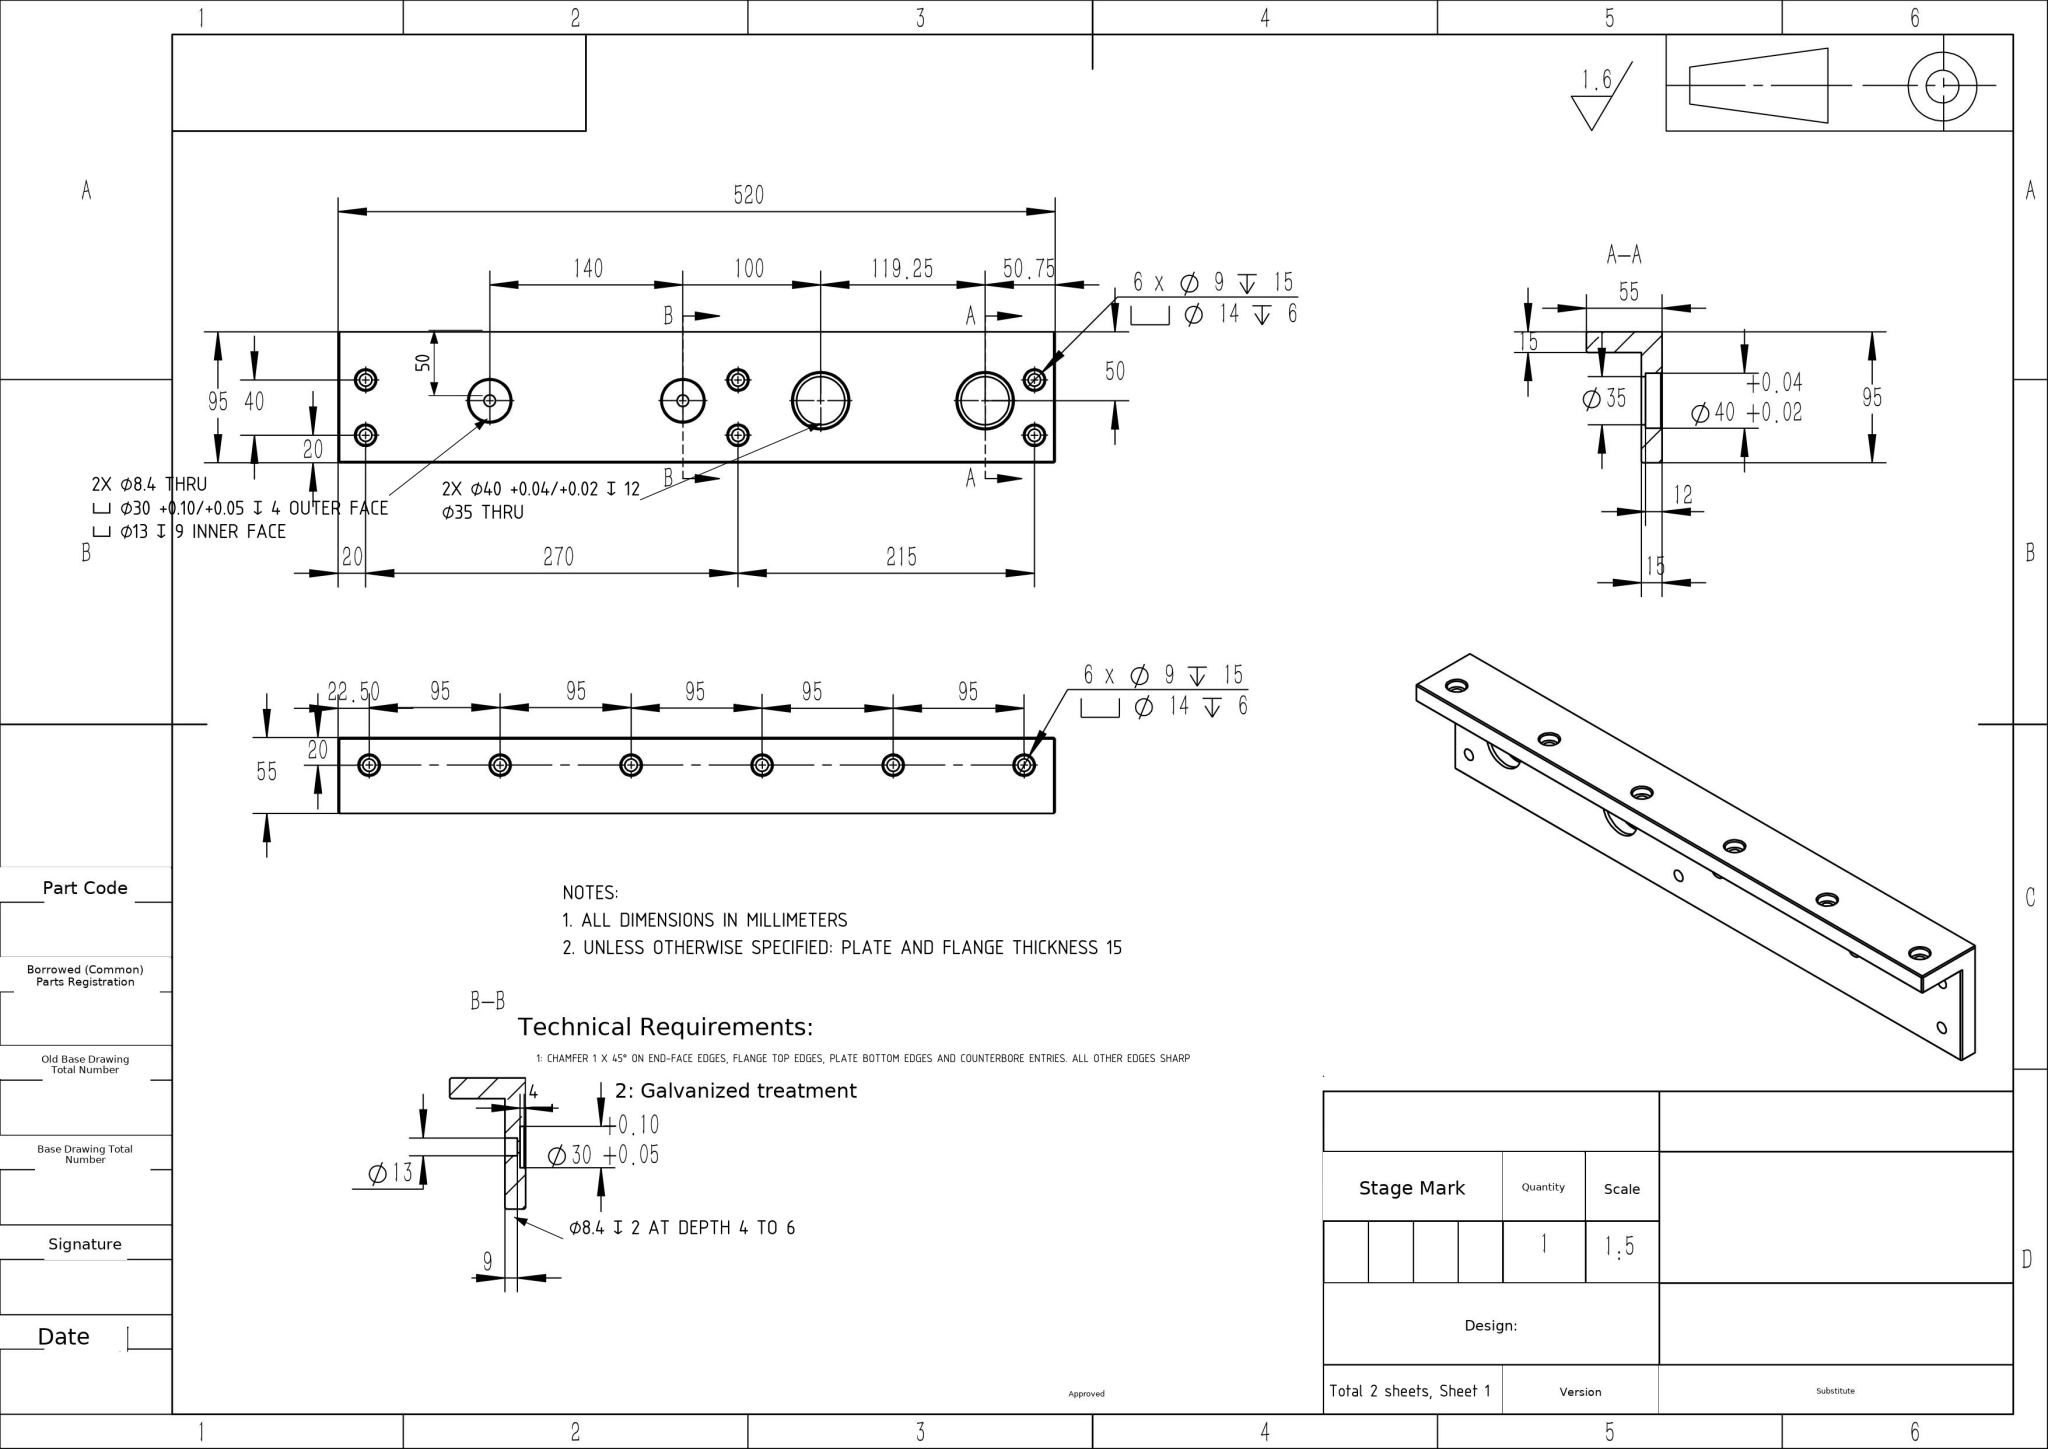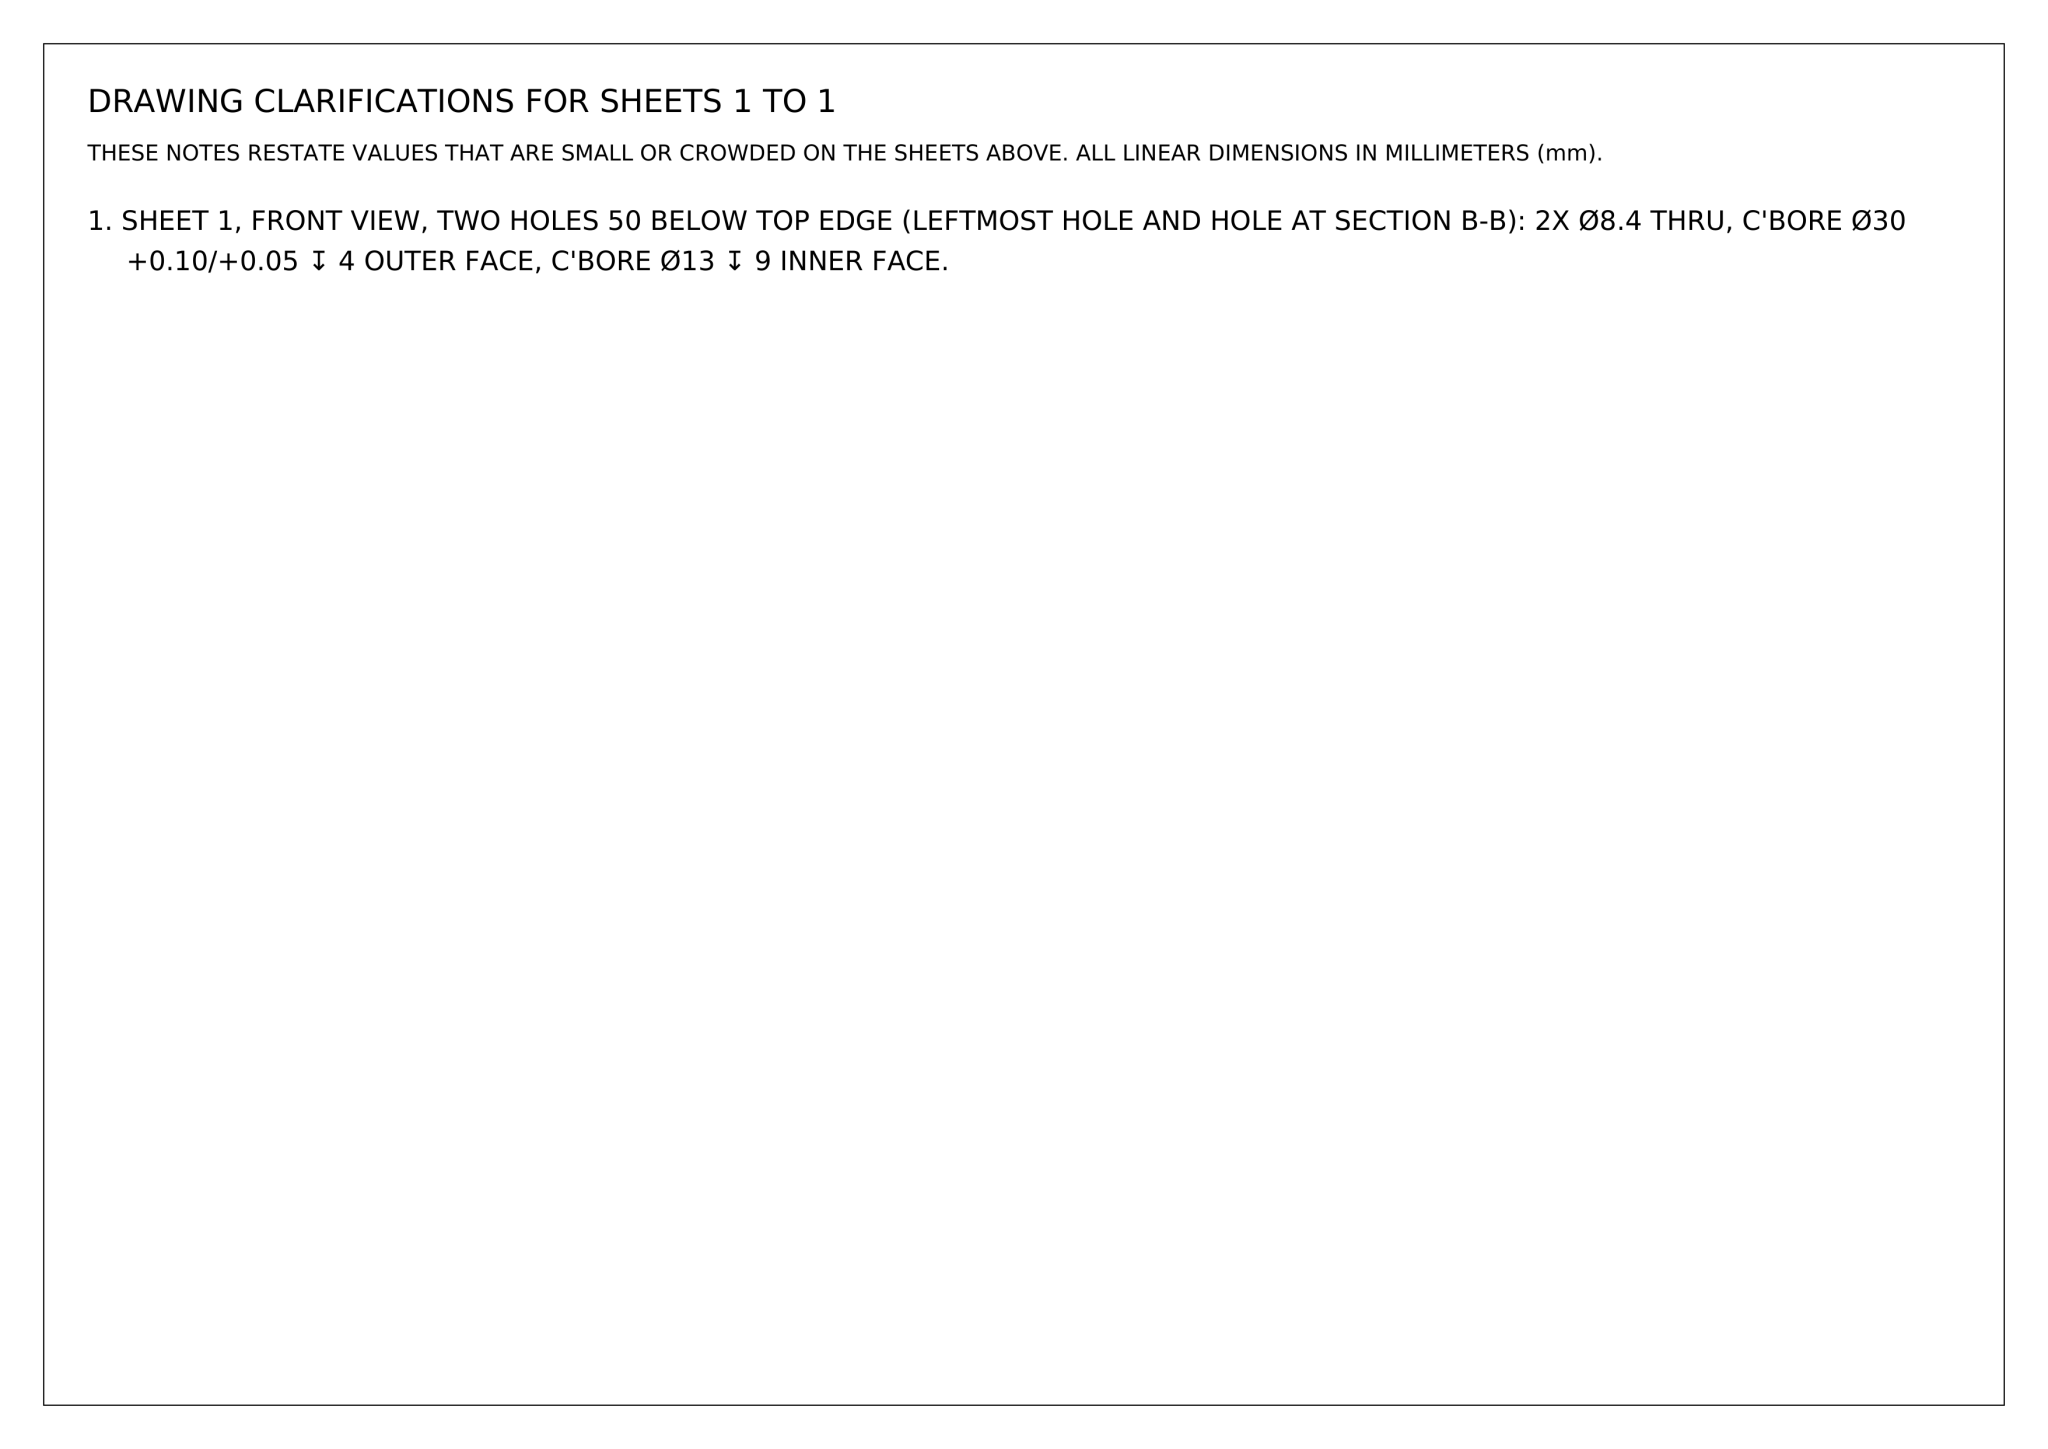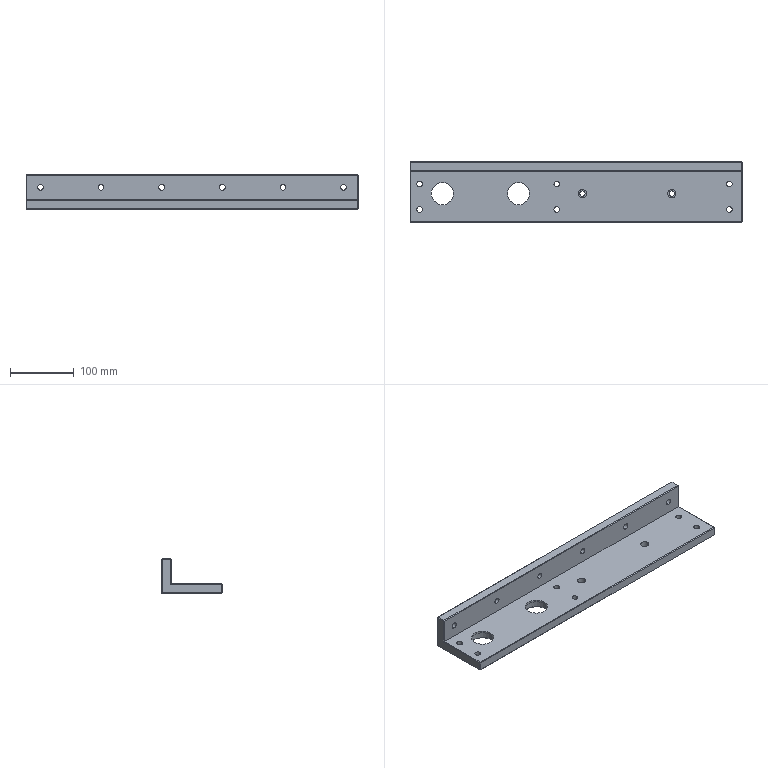Part | NX | mm | 1 solid | 150 faces | box 520 x 95 x 55 mm | volume 989013 mm3 | cylinder 68 | plane 50 | cone 32 | commonest cylinder face diameters 14 x24 9 x24 35 x4 40 x4 13 x4 8.4 x4 30 x4